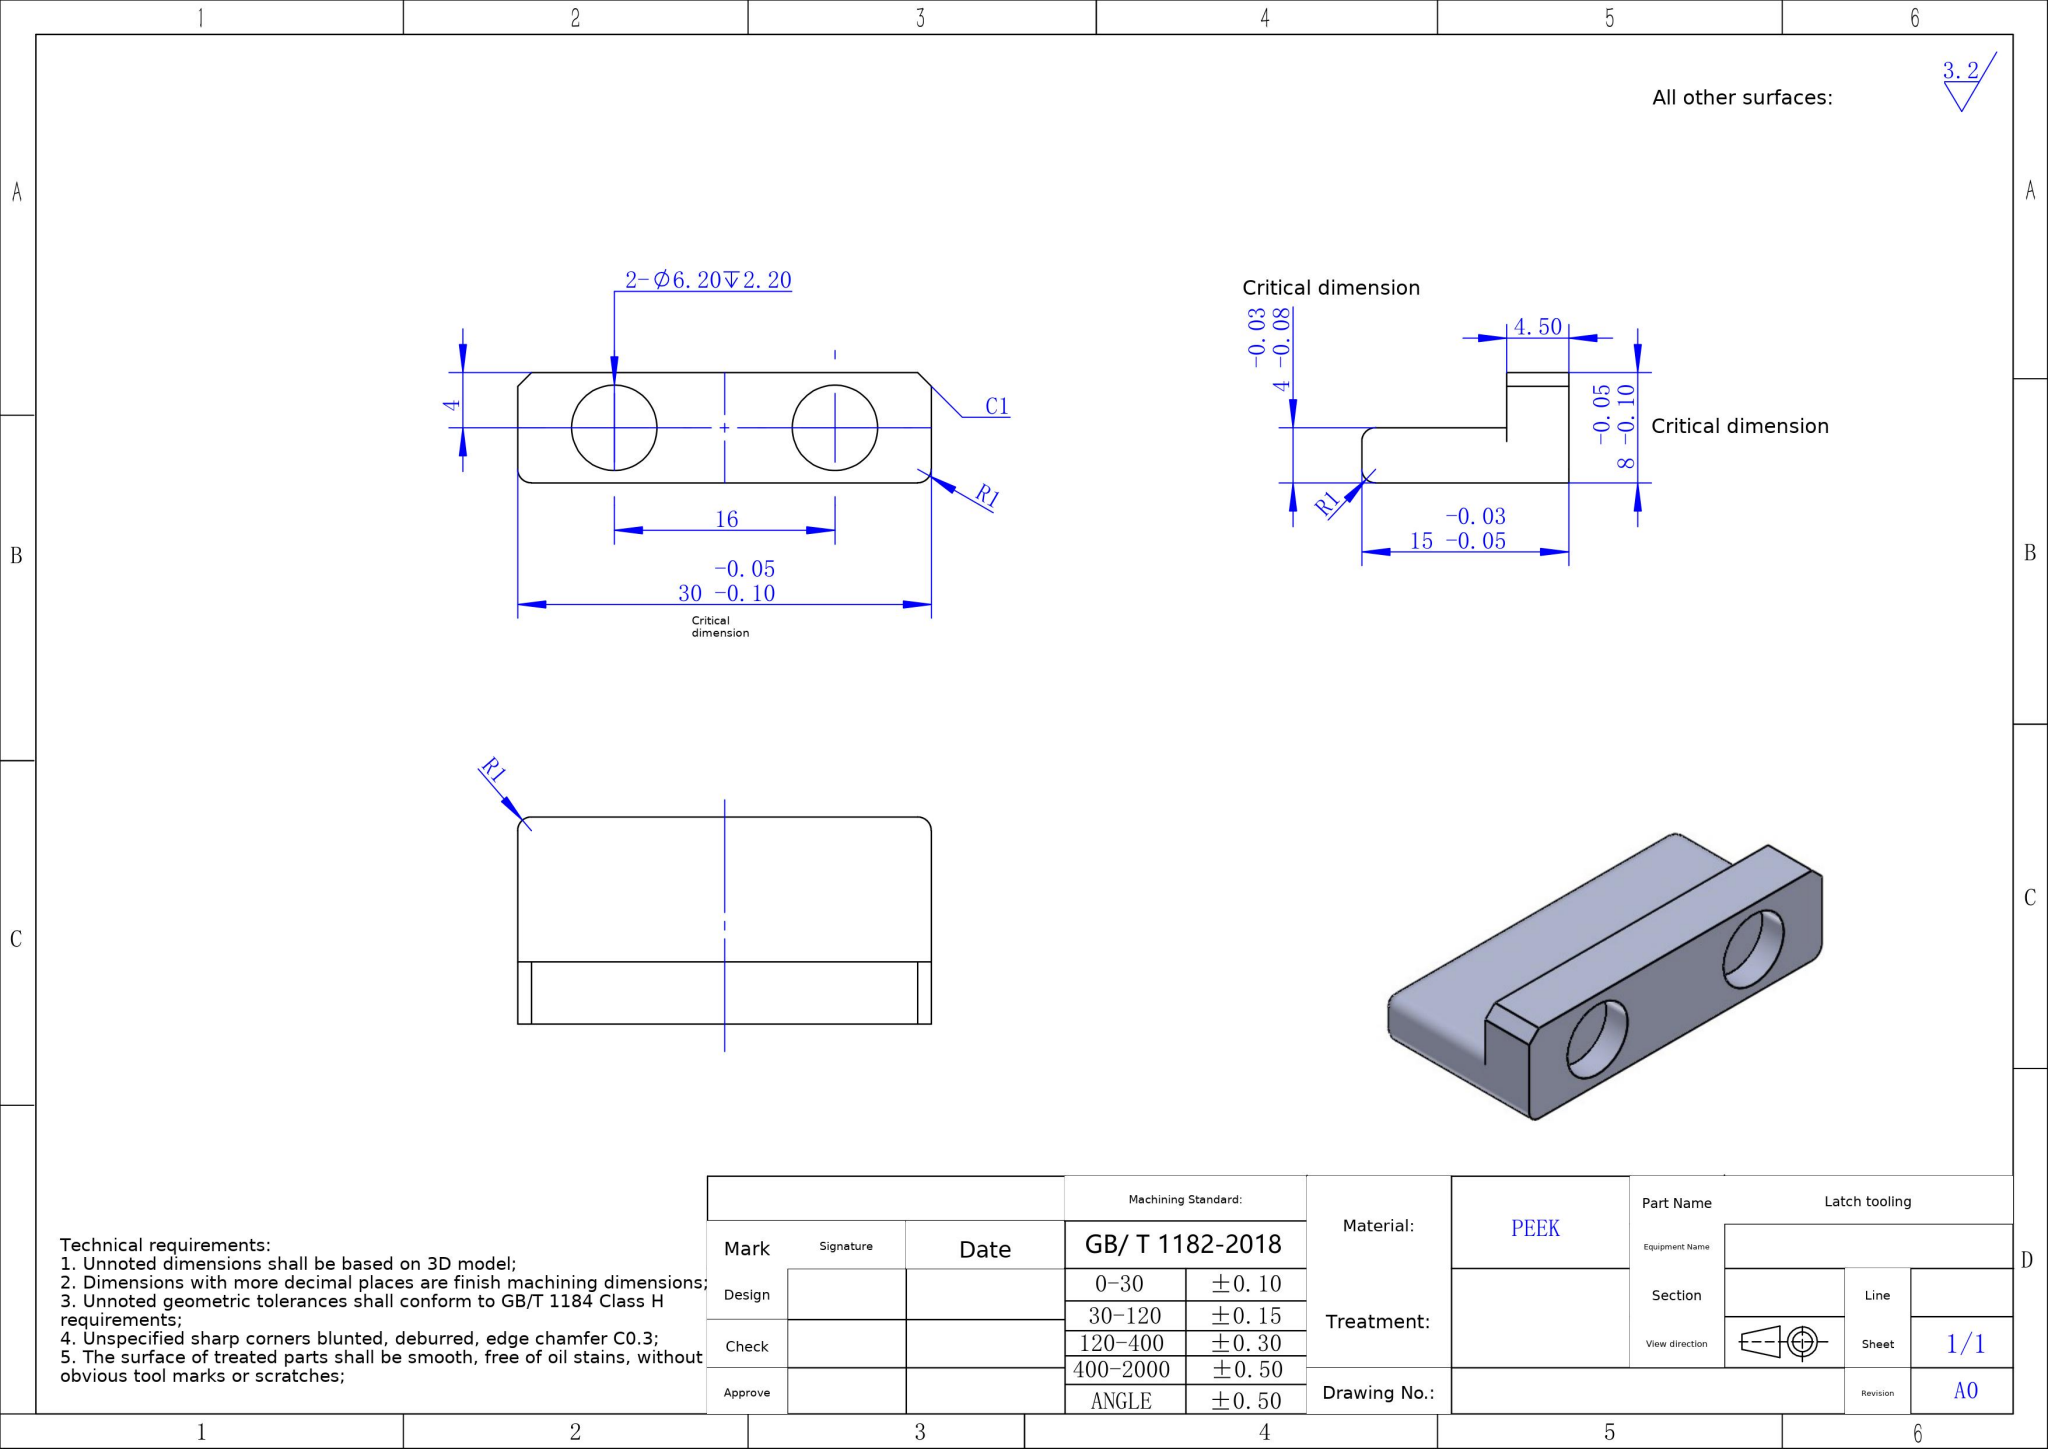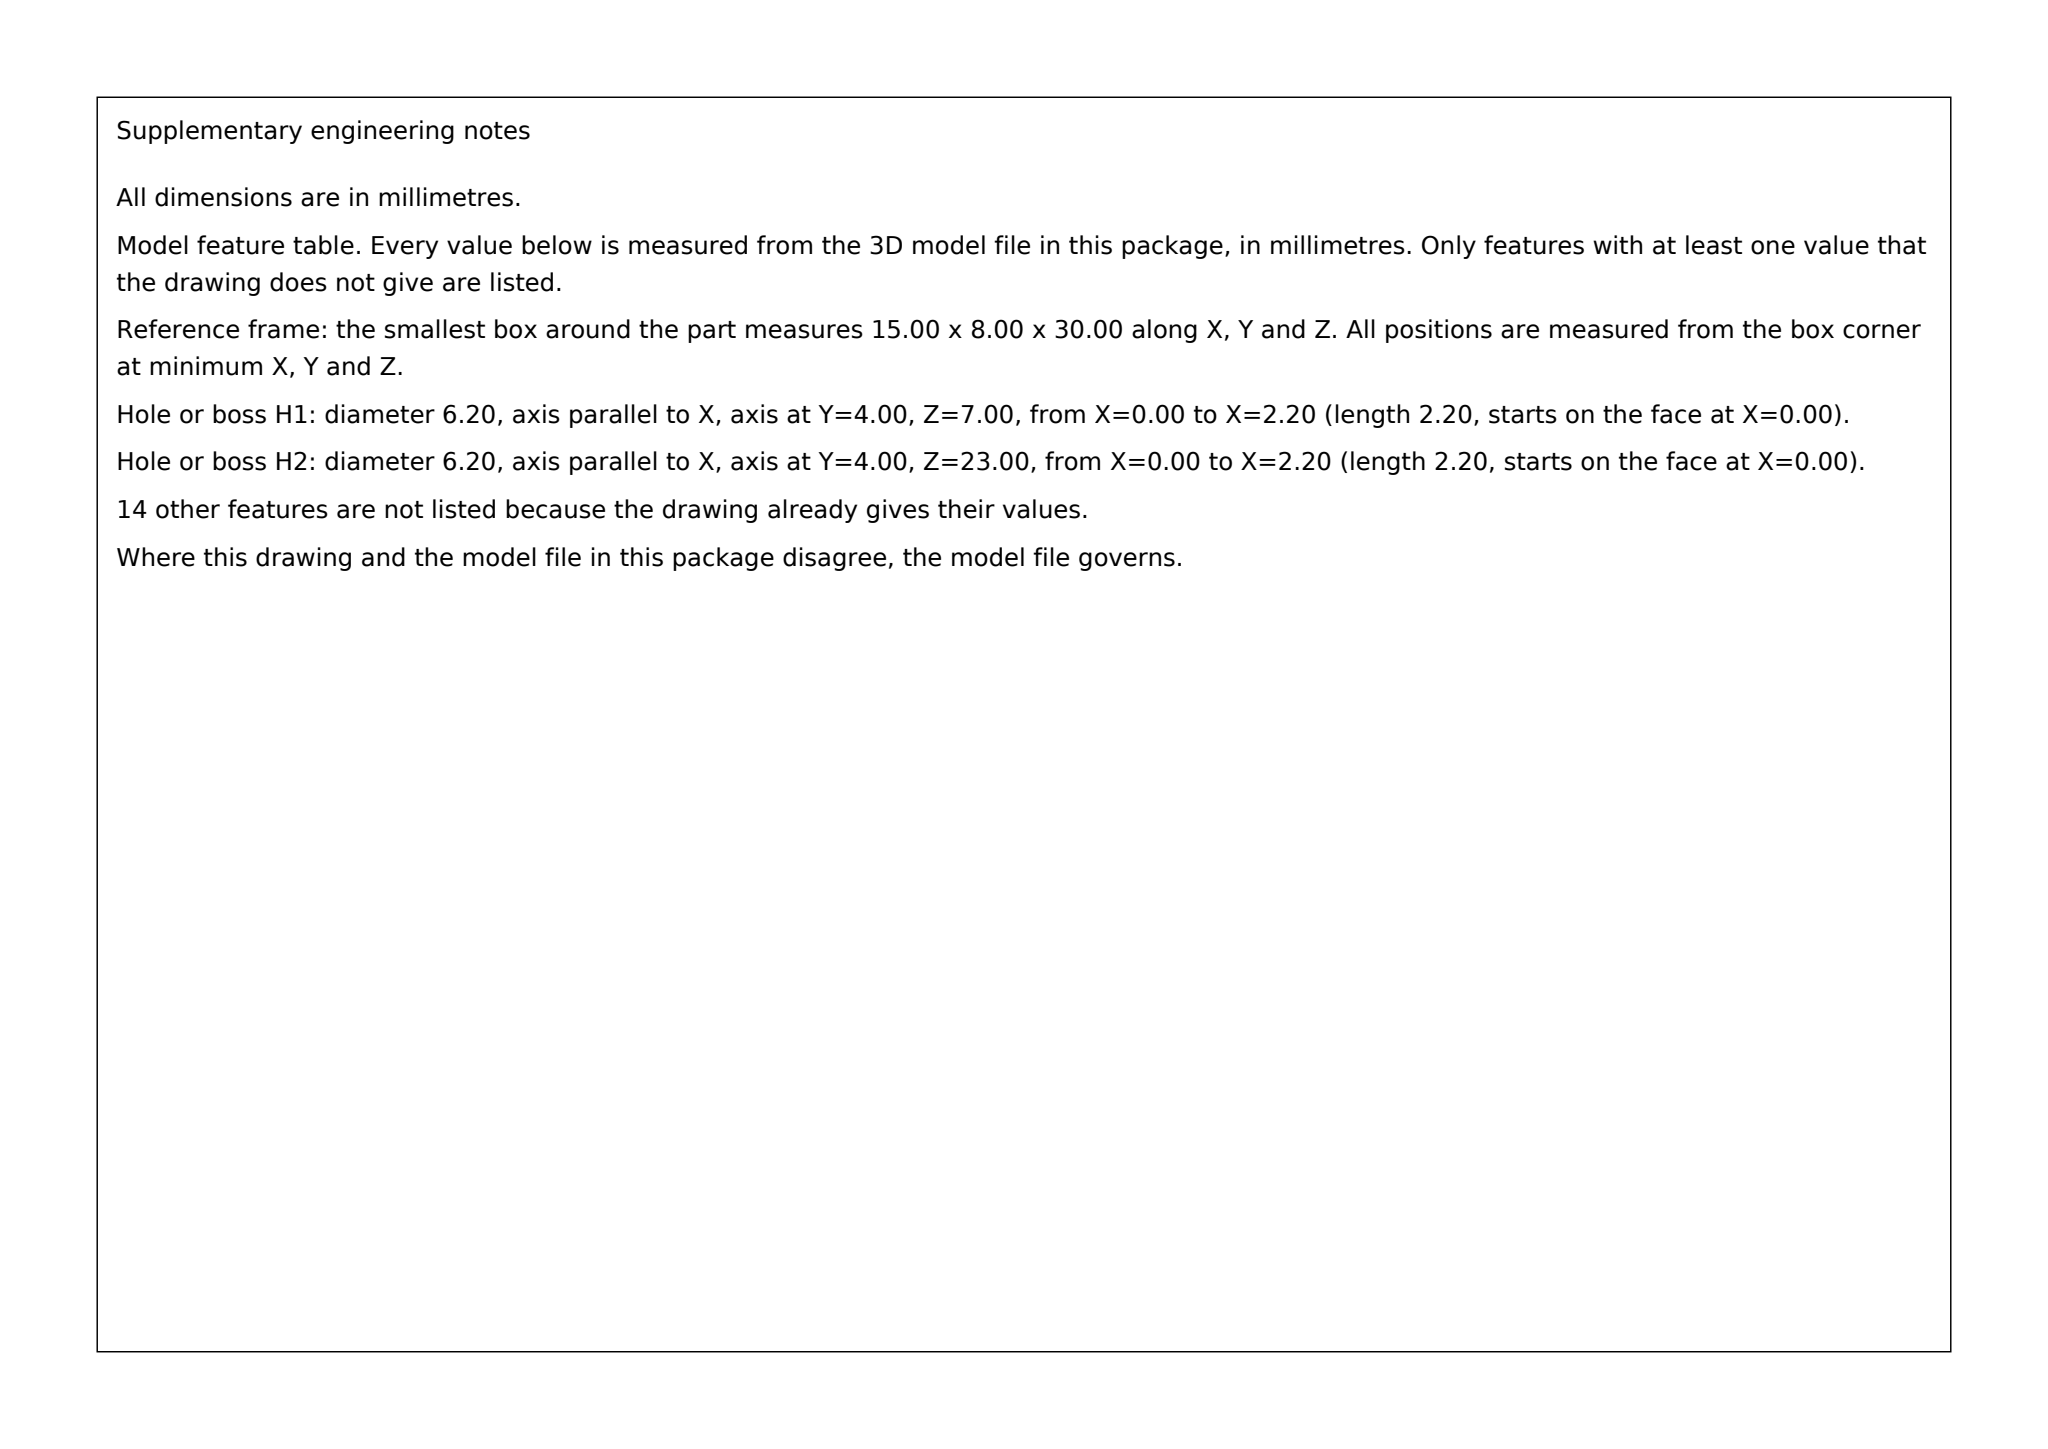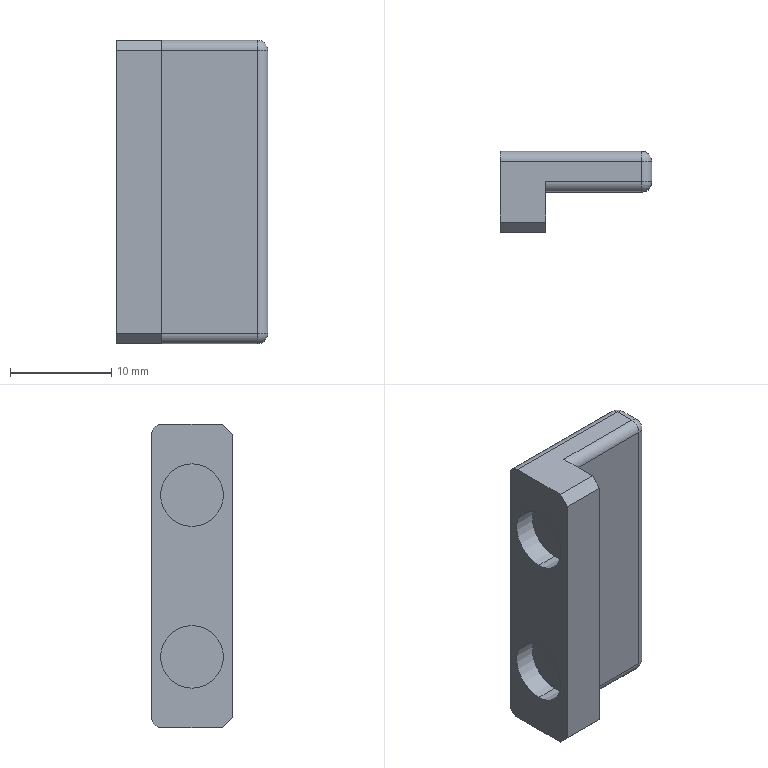Part | SolidWorks | mm | material PEEK | 1 solid | 28 faces | box 15 x 8 x 30 mm | volume 2178 mm3 | cylinder 12 | plane 12 | sphere 4 | commonest cylinder face diameters 2 x8 6.2 x4
build123d program:
from build123d import *

# Parameters (mm, degrees)
BOSS_EXTRUDE1_DEPTH = 15
SKETCH2_R           = 3.1
CUT_EXTRUDE1_DEPTH  = 2.2
CHAMFER1_SIZE       = 1
FILLET1_R           = 1


with BuildPart() as part:
    # Sketch1 → Boss-Extrude1 (new, symmetric)
    with BuildSketch(Plane.XY):
        Polygon((0, 0), (15, 0), (15, -4), (4.5, -4), (4.5, -8), (0, -8), align=None)
    extrude(amount=BOSS_EXTRUDE1_DEPTH, both=True)

    # Sketch2 → Cut-Extrude1 (cut)
    with BuildSketch(Plane.ZY):
        with Locations((8, -4)):
            Circle(SKETCH2_R)
        with Locations(Location((-8, -4, 0), (0, 0, 180))):
            Circle(SKETCH2_R)
    extrude(amount=-CUT_EXTRUDE1_DEPTH, mode=Mode.SUBTRACT)

    # Chamfer1
    chamfer1_edges = [part.edges().sort_by_distance(p)[0] for p in [
        (2.25, -8, -15),
        (2.25, -8, 15),
    ]]
    chamfer(chamfer1_edges, length=CHAMFER1_SIZE)

    # Fillet1
    fillet1_edges = [part.edges().sort_by_distance(p)[0] for p in [
        (15, 0, 0),
        (15, -4, 0),
        (9.75, -4, 15),
        (15, -2, 15),
        (7.5, 0, 15),
        (7.5, 0, -15),
        (15, -2, -15),
        (9.75, -4, -15),
    ]]
    fillet(fillet1_edges, radius=FILLET1_R)


solid = part.part
STEP:
#1=CARTESIAN_POINT('',(2.2,-4.,4.9));
#2=VERTEX_POINT('',#1);
#3=CARTESIAN_POINT('',(2.2,-4.,11.1));
#4=VERTEX_POINT('',#3);
#5=CARTESIAN_POINT('',(2.2,-4.,8.));
#6=DIRECTION('',(-1.,0.,0.));
#7=DIRECTION('',(0.,0.,1.));
#8=AXIS2_PLACEMENT_3D('',#5,#6,#7);
#9=CIRCLE('',#8,3.1);
#10=EDGE_CURVE('',#2,#4,#9,.T.);
#11=ORIENTED_EDGE('',*,*,#10,.F.);
#12=CARTESIAN_POINT('',(0.,-4.,4.9));
#13=VERTEX_POINT('',#12);
#14=CARTESIAN_POINT('',(2.2,-4.,4.9));
#15=DIRECTION('',(-1.,0.,0.));
#16=VECTOR('',#15,1000.);
#17=LINE('',#14,#16);
#18=EDGE_CURVE('',#2,#13,#17,.T.);
#19=ORIENTED_EDGE('',*,*,#18,.T.);
#20=CARTESIAN_POINT('',(0.,-4.,11.1));
#21=VERTEX_POINT('',#20);
#22=CARTESIAN_POINT('',(0.,-4.,8.));
#23=DIRECTION('',(-1.,0.,0.));
#24=DIRECTION('',(0.,0.,1.));
#25=AXIS2_PLACEMENT_3D('',#22,#23,#24);
#26=CIRCLE('',#25,3.1);
#27=EDGE_CURVE('',#13,#21,#26,.T.);
#28=ORIENTED_EDGE('',*,*,#27,.T.);
#29=CARTESIAN_POINT('',(2.2,-4.,11.1));
#30=DIRECTION('',(-1.,0.,0.));
#31=VECTOR('',#30,1000.);
#32=LINE('',#29,#31);
#33=EDGE_CURVE('',#4,#21,#32,.T.);
#34=ORIENTED_EDGE('',*,*,#33,.F.);
#35=EDGE_LOOP('',(#11,#19,#28,#34));
#36=FACE_OUTER_BOUND('',#35,.T.);
#37=CARTESIAN_POINT('',(2.2,-4.,8.));
#38=DIRECTION('',(-1.,0.,0.));
#39=DIRECTION('',(0.,0.,1.));
#40=AXIS2_PLACEMENT_3D('',#37,#38,#39);
#41=CYLINDRICAL_SURFACE('',#40,3.1);
#42=ADVANCED_FACE('',(#36),#41,.F.);
#43=CARTESIAN_POINT('',(2.2,-4.,-11.1));
#44=VERTEX_POINT('',#43);
#45=CARTESIAN_POINT('',(2.2,-4.,-4.9));
#46=VERTEX_POINT('',#45);
#47=CARTESIAN_POINT('',(2.2,-4.,-8.));
#48=DIRECTION('',(-1.,0.,0.));
#49=DIRECTION('',(0.,0.,-1.));
#50=AXIS2_PLACEMENT_3D('',#47,#48,#49);
#51=CIRCLE('',#50,3.1);
#52=EDGE_CURVE('',#44,#46,#51,.T.);
#53=ORIENTED_EDGE('',*,*,#52,.F.);
#54=CARTESIAN_POINT('',(0.,-4.,-11.1));
#55=VERTEX_POINT('',#54);
#56=CARTESIAN_POINT('',(2.2,-4.,-11.1));
#57=DIRECTION('',(-1.,0.,0.));
#58=VECTOR('',#57,1000.);
#59=LINE('',#56,#58);
#60=EDGE_CURVE('',#44,#55,#59,.T.);
#61=ORIENTED_EDGE('',*,*,#60,.T.);
#62=CARTESIAN_POINT('',(0.,-4.,-4.9));
#63=VERTEX_POINT('',#62);
#64=CARTESIAN_POINT('',(0.,-4.,-8.));
#65=DIRECTION('',(-1.,0.,0.));
#66=DIRECTION('',(0.,0.,-1.));
#67=AXIS2_PLACEMENT_3D('',#64,#65,#66);
#68=CIRCLE('',#67,3.1);
#69=EDGE_CURVE('',#55,#63,#68,.T.);
#70=ORIENTED_EDGE('',*,*,#69,.T.);
#71=CARTESIAN_POINT('',(2.2,-4.,-4.9));
#72=DIRECTION('',(-1.,0.,0.));
#73=VECTOR('',#72,1000.);
#74=LINE('',#71,#73);
#75=EDGE_CURVE('',#46,#63,#74,.T.);
#76=ORIENTED_EDGE('',*,*,#75,.F.);
#77=EDGE_LOOP('',(#53,#61,#70,#76));
#78=FACE_OUTER_BOUND('',#77,.T.);
#79=CARTESIAN_POINT('',(2.2,-4.,-8.));
#80=DIRECTION('',(-1.,0.,0.));
#81=DIRECTION('',(0.,0.,1.));
#82=AXIS2_PLACEMENT_3D('',#79,#80,#81);
#83=CYLINDRICAL_SURFACE('',#82,3.1);
#84=ADVANCED_FACE('',(#78),#83,.F.);
#85=CARTESIAN_POINT('',(0.,-4.,8.));
#86=DIRECTION('',(-1.,0.,0.));
#87=DIRECTION('',(0.,0.,1.));
#88=AXIS2_PLACEMENT_3D('',#85,#86,#87);
#89=CIRCLE('',#88,3.1);
#90=EDGE_CURVE('',#21,#13,#89,.T.);
#91=ORIENTED_EDGE('',*,*,#90,.F.);
#92=ORIENTED_EDGE('',*,*,#27,.F.);
#93=EDGE_LOOP('',(#91,#92));
#94=FACE_BOUND('',#93,.T.);
#95=CARTESIAN_POINT('',(0.,-4.,-8.));
#96=DIRECTION('',(-1.,0.,0.));
#97=DIRECTION('',(0.,0.,-1.));
#98=AXIS2_PLACEMENT_3D('',#95,#96,#97);
#99=CIRCLE('',#98,3.1);
#100=EDGE_CURVE('',#63,#55,#99,.T.);
#101=ORIENTED_EDGE('',*,*,#100,.F.);
#102=ORIENTED_EDGE('',*,*,#69,.F.);
#103=EDGE_LOOP('',(#101,#102));
#104=FACE_BOUND('',#103,.T.);
#105=CARTESIAN_POINT('',(0.,-1.,15.));
#106=VERTEX_POINT('',#105);
#107=CARTESIAN_POINT('',(0.,-7.,15.));
#108=VERTEX_POINT('',#107);
#109=CARTESIAN_POINT('',(0.,-8.,15.));
#110=DIRECTION('',(0.,-1.,0.));
#111=VECTOR('',#110,1000.);
#112=LINE('',#109,#111);
#113=EDGE_CURVE('',#106,#108,#112,.T.);
#114=ORIENTED_EDGE('',*,*,#113,.F.);
#115=CARTESIAN_POINT('',(0.,0.,14.));
#116=VERTEX_POINT('',#115);
#117=CARTESIAN_POINT('',(0.,-1.,14.));
#118=DIRECTION('',(-1.,0.,0.));
#119=DIRECTION('',(0.,0.,-1.));
#120=AXIS2_PLACEMENT_3D('',#117,#118,#119);
#121=CIRCLE('',#120,1.);
#122=EDGE_CURVE('',#106,#116,#121,.T.);
#123=ORIENTED_EDGE('',*,*,#122,.T.);
#124=CARTESIAN_POINT('',(0.,0.,-14.));
#125=VERTEX_POINT('',#124);
#126=CARTESIAN_POINT('',(0.,0.,15.));
#127=DIRECTION('',(0.,0.,-1.));
#128=VECTOR('',#127,1000.);
#129=LINE('',#126,#128);
#130=EDGE_CURVE('',#116,#125,#129,.T.);
#131=ORIENTED_EDGE('',*,*,#130,.T.);
#132=CARTESIAN_POINT('',(0.,-1.,-15.));
#133=VERTEX_POINT('',#132);
#134=CARTESIAN_POINT('',(0.,-1.,-14.));
#135=DIRECTION('',(-1.,0.,0.));
#136=DIRECTION('',(0.,0.,-1.));
#137=AXIS2_PLACEMENT_3D('',#134,#135,#136);
#138=CIRCLE('',#137,1.);
#139=EDGE_CURVE('',#125,#133,#138,.T.);
#140=ORIENTED_EDGE('',*,*,#139,.T.);
#141=CARTESIAN_POINT('',(0.,-7.,-15.));
#142=VERTEX_POINT('',#141);
#143=CARTESIAN_POINT('',(0.,-8.,-15.));
#144=DIRECTION('',(0.,-1.,0.));
#145=VECTOR('',#144,1000.);
#146=LINE('',#143,#145);
#147=EDGE_CURVE('',#133,#142,#146,.T.);
#148=ORIENTED_EDGE('',*,*,#147,.T.);
#149=CARTESIAN_POINT('',(0.,-8.,-14.));
#150=VERTEX_POINT('',#149);
#151=CARTESIAN_POINT('',(0.,-8.,-14.));
#152=DIRECTION('',(0.,-0.7071,0.7071));
#153=VECTOR('',#152,1000.);
#154=LINE('',#151,#153);
#155=EDGE_CURVE('',#142,#150,#154,.T.);
#156=ORIENTED_EDGE('',*,*,#155,.T.);
#157=CARTESIAN_POINT('',(0.,-8.,14.));
#158=VERTEX_POINT('',#157);
#159=CARTESIAN_POINT('',(0.,-8.,15.));
#160=DIRECTION('',(0.,0.,-1.));
#161=VECTOR('',#160,1000.);
#162=LINE('',#159,#161);
#163=EDGE_CURVE('',#158,#150,#162,.T.);
#164=ORIENTED_EDGE('',*,*,#163,.F.);
#165=CARTESIAN_POINT('',(0.,-7.,15.));
#166=DIRECTION('',(0.,0.7071,0.7071));
#167=VECTOR('',#166,1000.);
#168=LINE('',#165,#167);
#169=EDGE_CURVE('',#158,#108,#168,.T.);
#170=ORIENTED_EDGE('',*,*,#169,.T.);
#171=EDGE_LOOP('',(#114,#123,#131,#140,#148,#156,#164,#170));
#172=FACE_OUTER_BOUND('',#171,.T.);
#173=CARTESIAN_POINT('',(0.,-8.,15.));
#174=DIRECTION('',(1.,0.,0.));
#175=DIRECTION('',(0.,0.,-1.));
#176=AXIS2_PLACEMENT_3D('',#173,#174,#175);
#177=PLANE('',#176);
#178=ADVANCED_FACE('',(#94,#104,#172),#177,.F.);
#179=CARTESIAN_POINT('',(4.5,-8.,14.));
#180=VERTEX_POINT('',#179);
#181=CARTESIAN_POINT('',(4.5,-8.,-14.));
#182=VERTEX_POINT('',#181);
#183=CARTESIAN_POINT('',(4.5,-8.,15.));
#184=DIRECTION('',(0.,0.,-1.));
#185=VECTOR('',#184,1000.);
#186=LINE('',#183,#185);
#187=EDGE_CURVE('',#180,#182,#186,.T.);
#188=ORIENTED_EDGE('',*,*,#187,.F.);
#189=CARTESIAN_POINT('',(4.5,-8.,14.));
#190=DIRECTION('',(-1.,0.,0.));
#191=VECTOR('',#190,1000.);
#192=LINE('',#189,#191);
#193=EDGE_CURVE('',#180,#158,#192,.T.);
#194=ORIENTED_EDGE('',*,*,#193,.T.);
#195=ORIENTED_EDGE('',*,*,#163,.T.);
#196=CARTESIAN_POINT('',(4.5,-8.,-14.));
#197=DIRECTION('',(1.,0.,0.));
#198=VECTOR('',#197,1000.);
#199=LINE('',#196,#198);
#200=EDGE_CURVE('',#150,#182,#199,.T.);
#201=ORIENTED_EDGE('',*,*,#200,.T.);
#202=EDGE_LOOP('',(#188,#194,#195,#201));
#203=FACE_OUTER_BOUND('',#202,.T.);
#204=CARTESIAN_POINT('',(4.5,-8.,15.));
#205=DIRECTION('',(0.,1.,0.));
#206=DIRECTION('',(0.,0.,1.));
#207=AXIS2_PLACEMENT_3D('',#204,#205,#206);
#208=PLANE('',#207);
#209=ADVANCED_FACE('',(#203),#208,.F.);
#210=CARTESIAN_POINT('',(4.5,-7.,15.));
#211=VERTEX_POINT('',#210);
#212=CARTESIAN_POINT('',(4.5,-3.,15.));
#213=VERTEX_POINT('',#212);
#214=CARTESIAN_POINT('',(4.5,-4.,15.));
#215=DIRECTION('',(0.,1.,0.));
#216=VECTOR('',#215,1000.);
#217=LINE('',#214,#216);
#218=EDGE_CURVE('',#211,#213,#217,.T.);
#219=ORIENTED_EDGE('',*,*,#218,.F.);
#220=CARTESIAN_POINT('',(4.5,-7.,15.));
#221=DIRECTION('',(-0.,-0.7071,-0.7071));
#222=VECTOR('',#221,1000.);
#223=LINE('',#220,#222);
#224=EDGE_CURVE('',#211,#180,#223,.T.);
#225=ORIENTED_EDGE('',*,*,#224,.T.);
#226=ORIENTED_EDGE('',*,*,#187,.T.);
#227=CARTESIAN_POINT('',(4.5,-7.,-15.));
#228=VERTEX_POINT('',#227);
#229=CARTESIAN_POINT('',(4.5,-8.,-14.));
#230=DIRECTION('',(0.,0.7071,-0.7071));
#231=VECTOR('',#230,1000.);
#232=LINE('',#229,#231);
#233=EDGE_CURVE('',#182,#228,#232,.T.);
#234=ORIENTED_EDGE('',*,*,#233,.T.);
#235=CARTESIAN_POINT('',(4.5,-3.,-15.));
#236=VERTEX_POINT('',#235);
#237=CARTESIAN_POINT('',(4.5,-4.,-15.));
#238=DIRECTION('',(0.,1.,0.));
#239=VECTOR('',#238,1000.);
#240=LINE('',#237,#239);
#241=EDGE_CURVE('',#228,#236,#240,.T.);
#242=ORIENTED_EDGE('',*,*,#241,.T.);
#243=CARTESIAN_POINT('',(4.5,-4.,-14.));
#244=VERTEX_POINT('',#243);
#245=CARTESIAN_POINT('',(4.5,-3.,-14.));
#246=DIRECTION('',(-1.,0.,0.));
#247=DIRECTION('',(0.,-1.,0.));
#248=AXIS2_PLACEMENT_3D('',#245,#246,#247);
#249=CIRCLE('',#248,1.);
#250=EDGE_CURVE('',#236,#244,#249,.T.);
#251=ORIENTED_EDGE('',*,*,#250,.T.);
#252=CARTESIAN_POINT('',(4.5,-4.,14.));
#253=VERTEX_POINT('',#252);
#254=CARTESIAN_POINT('',(4.5,-4.,15.));
#255=DIRECTION('',(0.,0.,-1.));
#256=VECTOR('',#255,1000.);
#257=LINE('',#254,#256);
#258=EDGE_CURVE('',#253,#244,#257,.T.);
#259=ORIENTED_EDGE('',*,*,#258,.F.);
#260=CARTESIAN_POINT('',(4.5,-3.,14.));
#261=DIRECTION('',(-1.,0.,0.));
#262=DIRECTION('',(0.,-1.,0.));
#263=AXIS2_PLACEMENT_3D('',#260,#261,#262);
#264=CIRCLE('',#263,1.);
#265=EDGE_CURVE('',#253,#213,#264,.T.);
#266=ORIENTED_EDGE('',*,*,#265,.T.);
#267=EDGE_LOOP('',(#219,#225,#226,#234,#242,#251,#259,#266));
#268=FACE_OUTER_BOUND('',#267,.T.);
#269=CARTESIAN_POINT('',(4.5,-4.,15.));
#270=DIRECTION('',(-1.,0.,0.));
#271=DIRECTION('',(-0.,-1.,0.));
#272=AXIS2_PLACEMENT_3D('',#269,#270,#271);
#273=PLANE('',#272);
#274=ADVANCED_FACE('',(#268),#273,.F.);
#275=CARTESIAN_POINT('',(14.,-4.,-14.));
#276=VERTEX_POINT('',#275);
#277=CARTESIAN_POINT('',(14.,-4.,14.));
#278=VERTEX_POINT('',#277);
#279=CARTESIAN_POINT('',(14.,-4.,15.));
#280=DIRECTION('',(0.,0.,1.));
#281=VECTOR('',#280,1000.);
#282=LINE('',#279,#281);
#283=EDGE_CURVE('',#276,#278,#282,.T.);
#284=ORIENTED_EDGE('',*,*,#283,.T.);
#285=CARTESIAN_POINT('',(15.,-4.,14.));
#286=DIRECTION('',(-1.,-0.,0.));
#287=VECTOR('',#286,1000.);
#288=LINE('',#285,#287);
#289=EDGE_CURVE('',#278,#253,#288,.T.);
#290=ORIENTED_EDGE('',*,*,#289,.T.);
#291=ORIENTED_EDGE('',*,*,#258,.T.);
#292=CARTESIAN_POINT('',(15.,-4.,-14.));
#293=DIRECTION('',(1.,0.,0.));
#294=VECTOR('',#293,1000.);
#295=LINE('',#292,#294);
#296=EDGE_CURVE('',#244,#276,#295,.T.);
#297=ORIENTED_EDGE('',*,*,#296,.T.);
#298=EDGE_LOOP('',(#284,#290,#291,#297));
#299=FACE_OUTER_BOUND('',#298,.T.);
#300=CARTESIAN_POINT('',(15.,-4.,15.));
#301=DIRECTION('',(-0.,1.,0.));
#302=DIRECTION('',(-1.,-0.,0.));
#303=AXIS2_PLACEMENT_3D('',#300,#301,#302);
#304=PLANE('',#303);
#305=ADVANCED_FACE('',(#299),#304,.F.);
#306=CARTESIAN_POINT('',(15.,-3.,14.));
#307=VERTEX_POINT('',#306);
#308=CARTESIAN_POINT('',(15.,-3.,-14.));
#309=VERTEX_POINT('',#308);
#310=CARTESIAN_POINT('',(15.,-3.,15.));
#311=DIRECTION('',(0.,0.,-1.));
#312=VECTOR('',#311,1000.);
#313=LINE('',#310,#312);
#314=EDGE_CURVE('',#307,#309,#313,.T.);
#315=ORIENTED_EDGE('',*,*,#314,.T.);
#316=CARTESIAN_POINT('',(15.,-1.,-14.));
#317=VERTEX_POINT('',#316);
#318=CARTESIAN_POINT('',(15.,0.,-14.));
#319=DIRECTION('',(0.,1.,0.));
#320=VECTOR('',#319,1000.);
#321=LINE('',#318,#320);
#322=EDGE_CURVE('',#309,#317,#321,.T.);
#323=ORIENTED_EDGE('',*,*,#322,.T.);
#324=CARTESIAN_POINT('',(15.,-1.,14.));
#325=VERTEX_POINT('',#324);
#326=CARTESIAN_POINT('',(15.,-1.,15.));
#327=DIRECTION('',(0.,0.,1.));
#328=VECTOR('',#327,1000.);
#329=LINE('',#326,#328);
#330=EDGE_CURVE('',#317,#325,#329,.T.);
#331=ORIENTED_EDGE('',*,*,#330,.T.);
#332=CARTESIAN_POINT('',(15.,0.,14.));
#333=DIRECTION('',(0.,-1.,0.));
#334=VECTOR('',#333,1000.);
#335=LINE('',#332,#334);
#336=EDGE_CURVE('',#325,#307,#335,.T.);
#337=ORIENTED_EDGE('',*,*,#336,.T.);
#338=EDGE_LOOP('',(#315,#323,#331,#337));
#339=FACE_OUTER_BOUND('',#338,.T.);
#340=CARTESIAN_POINT('',(15.,0.,15.));
#341=DIRECTION('',(-1.,0.,0.));
#342=DIRECTION('',(0.,0.,1.));
#343=AXIS2_PLACEMENT_3D('',#340,#341,#342);
#344=PLANE('',#343);
#345=ADVANCED_FACE('',(#339),#344,.F.);
#346=ORIENTED_EDGE('',*,*,#130,.F.);
#347=CARTESIAN_POINT('',(14.,0.,14.));
#348=VERTEX_POINT('',#347);
#349=CARTESIAN_POINT('',(0.,0.,14.));
#350=DIRECTION('',(1.,0.,0.));
#351=VECTOR('',#350,1000.);
#352=LINE('',#349,#351);
#353=EDGE_CURVE('',#116,#348,#352,.T.);
#354=ORIENTED_EDGE('',*,*,#353,.T.);
#355=CARTESIAN_POINT('',(14.,0.,-14.));
#356=VERTEX_POINT('',#355);
#357=CARTESIAN_POINT('',(14.,0.,15.));
#358=DIRECTION('',(0.,0.,-1.));
#359=VECTOR('',#358,1000.);
#360=LINE('',#357,#359);
#361=EDGE_CURVE('',#348,#356,#360,.T.);
#362=ORIENTED_EDGE('',*,*,#361,.T.);
#363=CARTESIAN_POINT('',(0.,0.,-14.));
#364=DIRECTION('',(-1.,0.,0.));
#365=VECTOR('',#364,1000.);
#366=LINE('',#363,#365);
#367=EDGE_CURVE('',#356,#125,#366,.T.);
#368=ORIENTED_EDGE('',*,*,#367,.T.);
#369=EDGE_LOOP('',(#346,#354,#362,#368));
#370=FACE_OUTER_BOUND('',#369,.T.);
#371=CARTESIAN_POINT('',(0.,0.,15.));
#372=DIRECTION('',(0.,-1.,0.));
#373=DIRECTION('',(0.,0.,-1.));
#374=AXIS2_PLACEMENT_3D('',#371,#372,#373);
#375=PLANE('',#374);
#376=ADVANCED_FACE('',(#370),#375,.F.);
#377=CARTESIAN_POINT('',(14.,-3.,15.));
#378=VERTEX_POINT('',#377);
#379=CARTESIAN_POINT('',(14.,-1.,15.));
#380=VERTEX_POINT('',#379);
#381=CARTESIAN_POINT('',(14.,0.,15.));
#382=DIRECTION('',(0.,1.,0.));
#383=VECTOR('',#382,1000.);
#384=LINE('',#381,#383);
#385=EDGE_CURVE('',#378,#380,#384,.T.);
#386=ORIENTED_EDGE('',*,*,#385,.T.);
#387=CARTESIAN_POINT('',(0.,-1.,15.));
#388=DIRECTION('',(-1.,0.,0.));
#389=VECTOR('',#388,1000.);
#390=LINE('',#387,#389);
#391=EDGE_CURVE('',#380,#106,#390,.T.);
#392=ORIENTED_EDGE('',*,*,#391,.T.);
#393=ORIENTED_EDGE('',*,*,#113,.T.);
#394=CARTESIAN_POINT('',(0.,-7.,15.));
#395=DIRECTION('',(1.,0.,0.));
#396=VECTOR('',#395,1000.);
#397=LINE('',#394,#396);
#398=EDGE_CURVE('',#108,#211,#397,.T.);
#399=ORIENTED_EDGE('',*,*,#398,.T.);
#400=ORIENTED_EDGE('',*,*,#218,.T.);
#401=CARTESIAN_POINT('',(0.,-3.,15.));
#402=DIRECTION('',(1.,0.,0.));
#403=VECTOR('',#402,1000.);
#404=LINE('',#401,#403);
#405=EDGE_CURVE('',#213,#378,#404,.T.);
#406=ORIENTED_EDGE('',*,*,#405,.T.);
#407=EDGE_LOOP('',(#386,#392,#393,#399,#400,#406));
#408=FACE_OUTER_BOUND('',#407,.T.);
#409=CARTESIAN_POINT('',(0.,0.,15.));
#410=DIRECTION('',(0.,0.,-1.));
#411=DIRECTION('',(-1.,0.,0.));
#412=AXIS2_PLACEMENT_3D('',#409,#410,#411);
#413=PLANE('',#412);
#414=ADVANCED_FACE('',(#408),#413,.F.);
#415=ORIENTED_EDGE('',*,*,#147,.F.);
#416=CARTESIAN_POINT('',(14.,-1.,-15.));
#417=VERTEX_POINT('',#416);
#418=CARTESIAN_POINT('',(15.,-1.,-15.));
#419=DIRECTION('',(1.,0.,0.));
#420=VECTOR('',#419,1000.);
#421=LINE('',#418,#420);
#422=EDGE_CURVE('',#133,#417,#421,.T.);
#423=ORIENTED_EDGE('',*,*,#422,.T.);
#424=CARTESIAN_POINT('',(14.,-3.,-15.));
#425=VERTEX_POINT('',#424);
#426=CARTESIAN_POINT('',(14.,-4.,-15.));
#427=DIRECTION('',(0.,-1.,0.));
#428=VECTOR('',#427,1000.);
#429=LINE('',#426,#428);
#430=EDGE_CURVE('',#417,#425,#429,.T.);
#431=ORIENTED_EDGE('',*,*,#430,.T.);
#432=CARTESIAN_POINT('',(4.5,-3.,-15.));
#433=DIRECTION('',(-1.,-0.,0.));
#434=VECTOR('',#433,1000.);
#435=LINE('',#432,#434);
#436=EDGE_CURVE('',#425,#236,#435,.T.);
#437=ORIENTED_EDGE('',*,*,#436,.T.);
#438=ORIENTED_EDGE('',*,*,#241,.F.);
#439=CARTESIAN_POINT('',(0.,-7.,-15.));
#440=DIRECTION('',(-1.,0.,0.));
#441=VECTOR('',#440,1000.);
#442=LINE('',#439,#441);
#443=EDGE_CURVE('',#228,#142,#442,.T.);
#444=ORIENTED_EDGE('',*,*,#443,.T.);
#445=EDGE_LOOP('',(#415,#423,#431,#437,#438,#444));
#446=FACE_OUTER_BOUND('',#445,.T.);
#447=CARTESIAN_POINT('',(0.,0.,-15.));
#448=DIRECTION('',(0.,0.,-1.));
#449=DIRECTION('',(-1.,0.,0.));
#450=AXIS2_PLACEMENT_3D('',#447,#448,#449);
#451=PLANE('',#450);
#452=ADVANCED_FACE('',(#446),#451,.T.);
#453=ORIENTED_EDGE('',*,*,#60,.F.);
#454=CARTESIAN_POINT('',(2.2,-4.,-8.));
#455=DIRECTION('',(-1.,0.,0.));
#456=DIRECTION('',(0.,0.,-1.));
#457=AXIS2_PLACEMENT_3D('',#454,#455,#456);
#458=CIRCLE('',#457,3.1);
#459=EDGE_CURVE('',#46,#44,#458,.T.);
#460=ORIENTED_EDGE('',*,*,#459,.F.);
#461=ORIENTED_EDGE('',*,*,#75,.T.);
#462=ORIENTED_EDGE('',*,*,#100,.T.);
#463=EDGE_LOOP('',(#453,#460,#461,#462));
#464=FACE_OUTER_BOUND('',#463,.T.);
#465=CARTESIAN_POINT('',(2.2,-4.,-8.));
#466=DIRECTION('',(-1.,0.,0.));
#467=DIRECTION('',(0.,0.,1.));
#468=AXIS2_PLACEMENT_3D('',#465,#466,#467);
#469=CYLINDRICAL_SURFACE('',#468,3.1);
#470=ADVANCED_FACE('',(#464),#469,.F.);
#471=ORIENTED_EDGE('',*,*,#459,.T.);
#472=ORIENTED_EDGE('',*,*,#52,.T.);
#473=EDGE_LOOP('',(#471,#472));
#474=FACE_OUTER_BOUND('',#473,.T.);
#475=CARTESIAN_POINT('',(2.2,-4.,-8.));
#476=DIRECTION('',(1.,0.,0.));
#477=DIRECTION('',(0.,0.,-1.));
#478=AXIS2_PLACEMENT_3D('',#475,#476,#477);
#479=PLANE('',#478);
#480=ADVANCED_FACE('',(#474),#479,.F.);
#481=ORIENTED_EDGE('',*,*,#18,.F.);
#482=CARTESIAN_POINT('',(2.2,-4.,8.));
#483=DIRECTION('',(-1.,0.,0.));
#484=DIRECTION('',(0.,0.,1.));
#485=AXIS2_PLACEMENT_3D('',#482,#483,#484);
#486=CIRCLE('',#485,3.1);
#487=EDGE_CURVE('',#4,#2,#486,.T.);
#488=ORIENTED_EDGE('',*,*,#487,.F.);
#489=ORIENTED_EDGE('',*,*,#33,.T.);
#490=ORIENTED_EDGE('',*,*,#90,.T.);
#491=EDGE_LOOP('',(#481,#488,#489,#490));
#492=FACE_OUTER_BOUND('',#491,.T.);
#493=CARTESIAN_POINT('',(2.2,-4.,8.));
#494=DIRECTION('',(-1.,0.,0.));
#495=DIRECTION('',(0.,0.,1.));
#496=AXIS2_PLACEMENT_3D('',#493,#494,#495);
#497=CYLINDRICAL_SURFACE('',#496,3.1);
#498=ADVANCED_FACE('',(#492),#497,.F.);
#499=ORIENTED_EDGE('',*,*,#487,.T.);
#500=ORIENTED_EDGE('',*,*,#10,.T.);
#501=EDGE_LOOP('',(#499,#500));
#502=FACE_OUTER_BOUND('',#501,.T.);
#503=CARTESIAN_POINT('',(2.2,-4.,8.));
#504=DIRECTION('',(-1.,0.,0.));
#505=DIRECTION('',(0.,0.,1.));
#506=AXIS2_PLACEMENT_3D('',#503,#504,#505);
#507=PLANE('',#506);
#508=ADVANCED_FACE('',(#502),#507,.T.);
#509=ORIENTED_EDGE('',*,*,#169,.F.);
#510=ORIENTED_EDGE('',*,*,#193,.F.);
#511=ORIENTED_EDGE('',*,*,#224,.F.);
#512=ORIENTED_EDGE('',*,*,#398,.F.);
#513=EDGE_LOOP('',(#509,#510,#511,#512));
#514=FACE_OUTER_BOUND('',#513,.T.);
#515=CARTESIAN_POINT('',(0.,-7.,15.));
#516=DIRECTION('',(0.,0.7071,-0.7071));
#517=DIRECTION('',(1.,0.,0.));
#518=AXIS2_PLACEMENT_3D('',#515,#516,#517);
#519=PLANE('',#518);
#520=ADVANCED_FACE('',(#514),#519,.F.);
#521=ORIENTED_EDGE('',*,*,#155,.F.);
#522=ORIENTED_EDGE('',*,*,#443,.F.);
#523=ORIENTED_EDGE('',*,*,#233,.F.);
#524=ORIENTED_EDGE('',*,*,#200,.F.);
#525=EDGE_LOOP('',(#521,#522,#523,#524));
#526=FACE_OUTER_BOUND('',#525,.T.);
#527=CARTESIAN_POINT('',(4.5,-8.,-14.));
#528=DIRECTION('',(0.,-0.7071,-0.7071));
#529=DIRECTION('',(-1.,0.,0.));
#530=AXIS2_PLACEMENT_3D('',#527,#528,#529);
#531=PLANE('',#530);
#532=ADVANCED_FACE('',(#526),#531,.T.);
#533=ORIENTED_EDGE('',*,*,#122,.F.);
#534=ORIENTED_EDGE('',*,*,#391,.F.);
#535=CARTESIAN_POINT('',(14.,-1.,14.));
#536=DIRECTION('',(1.,0.,0.));
#537=DIRECTION('',(0.,0.,-1.));
#538=AXIS2_PLACEMENT_3D('',#535,#536,#537);
#539=CIRCLE('',#538,1.);
#540=EDGE_CURVE('',#348,#380,#539,.T.);
#541=ORIENTED_EDGE('',*,*,#540,.F.);
#542=ORIENTED_EDGE('',*,*,#353,.F.);
#543=EDGE_LOOP('',(#533,#534,#541,#542));
#544=FACE_OUTER_BOUND('',#543,.T.);
#545=CARTESIAN_POINT('',(0.,-1.,14.));
#546=DIRECTION('',(-1.,0.,0.));
#547=DIRECTION('',(0.,0.,1.));
#548=AXIS2_PLACEMENT_3D('',#545,#546,#547);
#549=CYLINDRICAL_SURFACE('',#548,1.);
#550=ADVANCED_FACE('',(#544),#549,.T.);
#551=CARTESIAN_POINT('',(14.,-1.,-14.));
#552=DIRECTION('',(0.,0.,-1.));
#553=DIRECTION('',(-1.,0.,0.));
#554=AXIS2_PLACEMENT_3D('',#551,#552,#553);
#555=CIRCLE('',#554,1.);
#556=EDGE_CURVE('',#356,#317,#555,.T.);
#557=ORIENTED_EDGE('',*,*,#556,.F.);
#558=ORIENTED_EDGE('',*,*,#361,.F.);
#559=CARTESIAN_POINT('',(14.,-1.,14.));
#560=DIRECTION('',(0.,0.,1.));
#561=DIRECTION('',(1.,0.,0.));
#562=AXIS2_PLACEMENT_3D('',#559,#560,#561);
#563=CIRCLE('',#562,1.);
#564=EDGE_CURVE('',#325,#348,#563,.T.);
#565=ORIENTED_EDGE('',*,*,#564,.F.);
#566=ORIENTED_EDGE('',*,*,#330,.F.);
#567=EDGE_LOOP('',(#557,#558,#565,#566));
#568=FACE_OUTER_BOUND('',#567,.T.);
#569=CARTESIAN_POINT('',(14.,-1.,15.));
#570=DIRECTION('',(0.,0.,-1.));
#571=DIRECTION('',(-1.,0.,0.));
#572=AXIS2_PLACEMENT_3D('',#569,#570,#571);
#573=CYLINDRICAL_SURFACE('',#572,1.);
#574=ADVANCED_FACE('',(#568),#573,.T.);
#575=ORIENTED_EDGE('',*,*,#139,.F.);
#576=ORIENTED_EDGE('',*,*,#367,.F.);
#577=CARTESIAN_POINT('',(14.,-1.,-14.));
#578=DIRECTION('',(1.,0.,0.));
#579=DIRECTION('',(0.,0.,-1.));
#580=AXIS2_PLACEMENT_3D('',#577,#578,#579);
#581=CIRCLE('',#580,1.);
#582=EDGE_CURVE('',#417,#356,#581,.T.);
#583=ORIENTED_EDGE('',*,*,#582,.F.);
#584=ORIENTED_EDGE('',*,*,#422,.F.);
#585=EDGE_LOOP('',(#575,#576,#583,#584));
#586=FACE_OUTER_BOUND('',#585,.T.);
#587=CARTESIAN_POINT('',(0.,-1.,-14.));
#588=DIRECTION('',(1.,0.,0.));
#589=DIRECTION('',(0.,0.,-1.));
#590=AXIS2_PLACEMENT_3D('',#587,#588,#589);
#591=CYLINDRICAL_SURFACE('',#590,1.);
#592=ADVANCED_FACE('',(#586),#591,.T.);
#593=ORIENTED_EDGE('',*,*,#564,.T.);
#594=ORIENTED_EDGE('',*,*,#540,.T.);
#595=CARTESIAN_POINT('',(14.,-1.,14.));
#596=DIRECTION('',(0.,-1.,0.));
#597=DIRECTION('',(0.,0.,1.));
#598=AXIS2_PLACEMENT_3D('',#595,#596,#597);
#599=CIRCLE('',#598,1.);
#600=EDGE_CURVE('',#325,#380,#599,.T.);
#601=ORIENTED_EDGE('',*,*,#600,.F.);
#602=EDGE_LOOP('',(#593,#594,#601));
#603=FACE_OUTER_BOUND('',#602,.T.);
#604=CARTESIAN_POINT('',(14.,-1.,14.));
#605=DIRECTION('',(0.,1.,0.));
#606=DIRECTION('',(1.,0.,0.));
#607=AXIS2_PLACEMENT_3D('',#604,#605,#606);
#608=SPHERICAL_SURFACE('',#607,1.);
#609=ADVANCED_FACE('',(#603),#608,.T.);
#610=ORIENTED_EDGE('',*,*,#582,.T.);
#611=ORIENTED_EDGE('',*,*,#556,.T.);
#612=CARTESIAN_POINT('',(14.,-1.,-14.));
#613=DIRECTION('',(0.,-1.,0.));
#614=DIRECTION('',(0.,0.,1.));
#615=AXIS2_PLACEMENT_3D('',#612,#613,#614);
#616=CIRCLE('',#615,1.);
#617=EDGE_CURVE('',#417,#317,#616,.T.);
#618=ORIENTED_EDGE('',*,*,#617,.F.);
#619=EDGE_LOOP('',(#610,#611,#618));
#620=FACE_OUTER_BOUND('',#619,.T.);
#621=CARTESIAN_POINT('',(14.,-1.,-14.));
#622=DIRECTION('',(0.,1.,0.));
#623=DIRECTION('',(1.,0.,0.));
#624=AXIS2_PLACEMENT_3D('',#621,#622,#623);
#625=SPHERICAL_SURFACE('',#624,1.);
#626=ADVANCED_FACE('',(#620),#625,.T.);
#627=ORIENTED_EDGE('',*,*,#265,.F.);
#628=ORIENTED_EDGE('',*,*,#289,.F.);
#629=CARTESIAN_POINT('',(14.,-3.,14.));
#630=DIRECTION('',(1.,0.,0.));
#631=DIRECTION('',(0.,0.,-1.));
#632=AXIS2_PLACEMENT_3D('',#629,#630,#631);
#633=CIRCLE('',#632,1.);
#634=EDGE_CURVE('',#378,#278,#633,.T.);
#635=ORIENTED_EDGE('',*,*,#634,.F.);
#636=ORIENTED_EDGE('',*,*,#405,.F.);
#637=EDGE_LOOP('',(#627,#628,#635,#636));
#638=FACE_OUTER_BOUND('',#637,.T.);
#639=CARTESIAN_POINT('',(0.,-3.,14.));
#640=DIRECTION('',(1.,0.,0.));
#641=DIRECTION('',(-0.,1.,0.));
#642=AXIS2_PLACEMENT_3D('',#639,#640,#641);
#643=CYLINDRICAL_SURFACE('',#642,1.);
#644=ADVANCED_FACE('',(#638),#643,.T.);
#645=ORIENTED_EDGE('',*,*,#600,.T.);
#646=ORIENTED_EDGE('',*,*,#385,.F.);
#647=CARTESIAN_POINT('',(14.,-3.,14.));
#648=DIRECTION('',(0.,-1.,0.));
#649=DIRECTION('',(0.,0.,-1.));
#650=AXIS2_PLACEMENT_3D('',#647,#648,#649);
#651=CIRCLE('',#650,1.);
#652=EDGE_CURVE('',#307,#378,#651,.T.);
#653=ORIENTED_EDGE('',*,*,#652,.F.);
#654=ORIENTED_EDGE('',*,*,#336,.F.);
#655=EDGE_LOOP('',(#645,#646,#653,#654));
#656=FACE_OUTER_BOUND('',#655,.T.);
#657=CARTESIAN_POINT('',(14.,0.,14.));
#658=DIRECTION('',(0.,1.,0.));
#659=DIRECTION('',(0.,0.,1.));
#660=AXIS2_PLACEMENT_3D('',#657,#658,#659);
#661=CYLINDRICAL_SURFACE('',#660,1.);
#662=ADVANCED_FACE('',(#656),#661,.T.);
#663=ORIENTED_EDGE('',*,*,#617,.T.);
#664=ORIENTED_EDGE('',*,*,#322,.F.);
#665=CARTESIAN_POINT('',(14.,-3.,-14.));
#666=DIRECTION('',(0.,-1.,0.));
#667=DIRECTION('',(0.,0.,-1.));
#668=AXIS2_PLACEMENT_3D('',#665,#666,#667);
#669=CIRCLE('',#668,1.);
#670=EDGE_CURVE('',#425,#309,#669,.T.);
#671=ORIENTED_EDGE('',*,*,#670,.F.);
#672=ORIENTED_EDGE('',*,*,#430,.F.);
#673=EDGE_LOOP('',(#663,#664,#671,#672));
#674=FACE_OUTER_BOUND('',#673,.T.);
#675=CARTESIAN_POINT('',(14.,0.,-14.));
#676=DIRECTION('',(0.,-1.,0.));
#677=DIRECTION('',(0.,0.,-1.));
#678=AXIS2_PLACEMENT_3D('',#675,#676,#677);
#679=CYLINDRICAL_SURFACE('',#678,1.);
#680=ADVANCED_FACE('',(#674),#679,.T.);
#681=ORIENTED_EDGE('',*,*,#250,.F.);
#682=ORIENTED_EDGE('',*,*,#436,.F.);
#683=CARTESIAN_POINT('',(14.,-3.,-14.));
#684=DIRECTION('',(1.,0.,0.));
#685=DIRECTION('',(0.,0.,-1.));
#686=AXIS2_PLACEMENT_3D('',#683,#684,#685);
#687=CIRCLE('',#686,1.);
#688=EDGE_CURVE('',#276,#425,#687,.T.);
#689=ORIENTED_EDGE('',*,*,#688,.F.);
#690=ORIENTED_EDGE('',*,*,#296,.F.);
#691=EDGE_LOOP('',(#681,#682,#689,#690));
#692=FACE_OUTER_BOUND('',#691,.T.);
#693=CARTESIAN_POINT('',(15.,-3.,-14.));
#694=DIRECTION('',(-1.,-0.,0.));
#695=DIRECTION('',(0.,-1.,0.));
#696=AXIS2_PLACEMENT_3D('',#693,#694,#695);
#697=CYLINDRICAL_SURFACE('',#696,1.);
#698=ADVANCED_FACE('',(#692),#697,.T.);
#699=ORIENTED_EDGE('',*,*,#652,.T.);
#700=ORIENTED_EDGE('',*,*,#634,.T.);
#701=CARTESIAN_POINT('',(14.,-3.,14.));
#702=DIRECTION('',(0.,0.,-1.));
#703=DIRECTION('',(1.,0.,0.));
#704=AXIS2_PLACEMENT_3D('',#701,#702,#703);
#705=CIRCLE('',#704,1.);
#706=EDGE_CURVE('',#307,#278,#705,.T.);
#707=ORIENTED_EDGE('',*,*,#706,.F.);
#708=EDGE_LOOP('',(#699,#700,#707));
#709=FACE_OUTER_BOUND('',#708,.T.);
#710=CARTESIAN_POINT('',(14.,-3.,14.));
#711=DIRECTION('',(0.,1.,0.));
#712=DIRECTION('',(1.,0.,0.));
#713=AXIS2_PLACEMENT_3D('',#710,#711,#712);
#714=SPHERICAL_SURFACE('',#713,1.);
#715=ADVANCED_FACE('',(#709),#714,.T.);
#716=ORIENTED_EDGE('',*,*,#688,.T.);
#717=ORIENTED_EDGE('',*,*,#670,.T.);
#718=CARTESIAN_POINT('',(14.,-3.,-14.));
#719=DIRECTION('',(0.,0.,1.));
#720=DIRECTION('',(-1.,0.,0.));
#721=AXIS2_PLACEMENT_3D('',#718,#719,#720);
#722=CIRCLE('',#721,1.);
#723=EDGE_CURVE('',#276,#309,#722,.T.);
#724=ORIENTED_EDGE('',*,*,#723,.F.);
#725=EDGE_LOOP('',(#716,#717,#724));
#726=FACE_OUTER_BOUND('',#725,.T.);
#727=CARTESIAN_POINT('',(14.,-3.,-14.));
#728=DIRECTION('',(0.,1.,0.));
#729=DIRECTION('',(1.,0.,0.));
#730=AXIS2_PLACEMENT_3D('',#727,#728,#729);
#731=SPHERICAL_SURFACE('',#730,1.);
#732=ADVANCED_FACE('',(#726),#731,.T.);
#733=ORIENTED_EDGE('',*,*,#706,.T.);
#734=ORIENTED_EDGE('',*,*,#283,.F.);
#735=ORIENTED_EDGE('',*,*,#723,.T.);
#736=ORIENTED_EDGE('',*,*,#314,.F.);
#737=EDGE_LOOP('',(#733,#734,#735,#736));
#738=FACE_OUTER_BOUND('',#737,.T.);
#739=CARTESIAN_POINT('',(14.,-3.,15.));
#740=DIRECTION('',(0.,0.,-1.));
#741=DIRECTION('',(-1.,0.,0.));
#742=AXIS2_PLACEMENT_3D('',#739,#740,#741);
#743=CYLINDRICAL_SURFACE('',#742,1.);
#744=ADVANCED_FACE('',(#738),#743,.T.);
#745=CLOSED_SHELL('',(#42,#84,#178,#209,#274,#305,#345,#376,#414,#452,#470,#480,#498,#508,#520,#532,#550,#574,#592,#609,#626,#644,#662,#680,#698,#715,#732,#744));
#746=MANIFOLD_SOLID_BREP('',#745);
#747=CARTESIAN_POINT('',(0.,0.,0.));
#748=DIRECTION('',(0.,0.,1.));
#749=DIRECTION('',(1.,0.,0.));
#750=AXIS2_PLACEMENT_3D('',#747,#748,#749);
#751=(LENGTH_UNIT()NAMED_UNIT(*)SI_UNIT(.MILLI.,.METRE.));
#752=UNCERTAINTY_MEASURE_WITH_UNIT(LENGTH_MEASURE(0.00001),#751,'','');
#753=(NAMED_UNIT(*)PLANE_ANGLE_UNIT()SI_UNIT($,.RADIAN.));
#754=(NAMED_UNIT(*)SI_UNIT($,.STERADIAN.)SOLID_ANGLE_UNIT());
#755=(GEOMETRIC_REPRESENTATION_CONTEXT(3)GLOBAL_UNCERTAINTY_ASSIGNED_CONTEXT((#752))GLOBAL_UNIT_ASSIGNED_CONTEXT((#751,#753,#754))REPRESENTATION_CONTEXT('',''));
#756=ADVANCED_BREP_SHAPE_REPRESENTATION('',(#746,#750),#755);